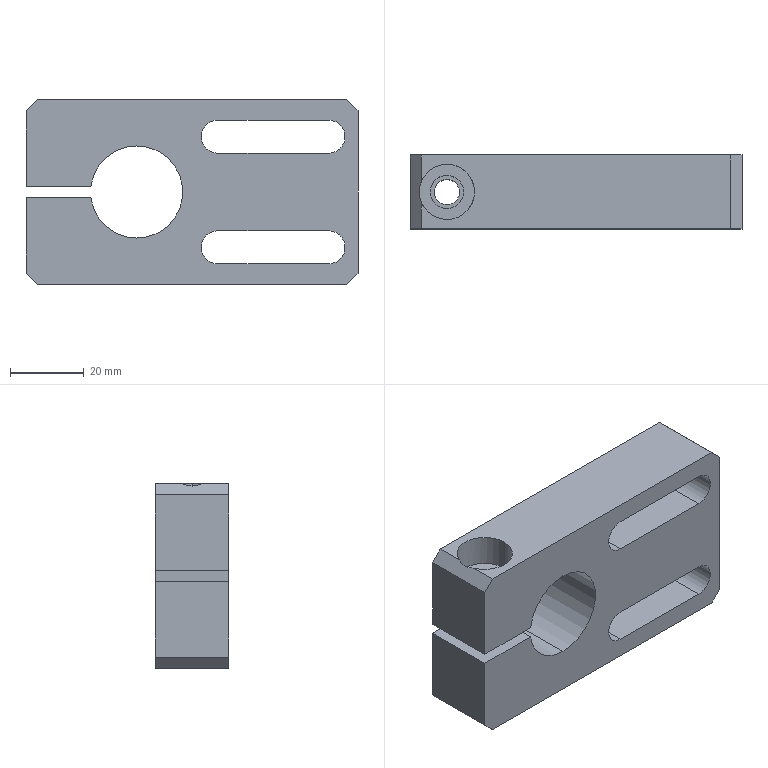Component | SolidWorks | 8TC-A15004-90-01A-1 | 1 solid | 31 faces | box 90 x 20 x 50 mm | volume 62105 mm3 | plane 18 | cylinder 13 | commonest cylinder face diameters 9 x6 25 x3 6.8 x2 15 x2 | material A3
build123d program:
from build123d import *

# Parameters (mm, degrees)
SKETCH1_W                                       = 90
SKETCH1_H                                       = 50
BOSS_EXTRUDE1_DEPTH                             = 10
SKETCH2_R                                       = 12.5
CUT_EXTRUDE1_DEPTH                              = 56.227
CHAMFER1_SIZE                                   = 3
CUT_EXTRUDE2_DEPTH                              = 56.227
SKETCH4_W                                       = 17.59
SKETCH4_H                                       = 3
CUT_EXTRUDE3_DEPTH                              = 56.227
M8_HEX_SOCKET_HEAD_CAP_SCREW_CBORE1_D           = 9
M8_HEX_SOCKET_HEAD_CAP_SCREW_CBORE1_DEPTH       = 23.5
M8_HEX_SOCKET_HEAD_CAP_SCREW_CBORE1_CBORE_D     = 15
M8_HEX_SOCKET_HEAD_CAP_SCREW_CBORE1_CBORE_DEPTH = 8.6
M8_TAPPED_HOLE1_D                               = 6.8


with BuildPart() as part:
    # Sketch1 → Boss-Extrude1 (new, symmetric)
    with BuildSketch(Plane(origin=(0, 0, 0), x_dir=(1, 0, 0), z_dir=(0, 1, 0))):
        Rectangle(SKETCH1_W, SKETCH1_H)
    extrude(amount=BOSS_EXTRUDE1_DEPTH, both=True)

    # Sketch2 → Cut-Extrude1 (cut, through all)
    with BuildSketch(Plane(origin=(0, 10, 0), x_dir=(1, 0, 0), z_dir=(0, 1, 0))):
        with Locations(Location((-15, 0, 0), (0, 0, 270))):
            Circle(SKETCH2_R)
    extrude(amount=-CUT_EXTRUDE1_DEPTH, mode=Mode.SUBTRACT)

    # Chamfer1
    chamfer1_edges = [part.edges().sort_by_distance(p)[0] for p in [
        (45, 0, 25),
        (-45, 0, 25),
        (-45, 0, -25),
        (45, 0, -25),
    ]]
    chamfer(chamfer1_edges, length=CHAMFER1_SIZE)

    # Sketch3 → Cut-Extrude2 (cut, through all)
    with BuildSketch(Plane(origin=(0, 10, 0), x_dir=(1, 0, 0), z_dir=(0, 1, 0))):
        with BuildLine():
            Line((7, 19.5), (37, 19.5))
            ThreePointArc((37, 19.5), (41.5, 15), (37, 10.5))
            Line((37, 10.5), (7, 10.5))
            ThreePointArc((7, 10.5), (2.5, 15), (7, 19.5))
        make_face()
        with BuildLine():
            Line((7, -19.5), (37, -19.5))
            ThreePointArc((37, -19.5), (41.5, -15), (37, -10.5))
            Line((37, -10.5), (7, -10.5))
            ThreePointArc((7, -10.5), (2.5, -15), (7, -19.5))
        make_face()
    extrude(amount=-CUT_EXTRUDE2_DEPTH, mode=Mode.SUBTRACT)

    # Sketch4 → Cut-Extrude3 (cut, through all)
    with BuildSketch(Plane(origin=(0, 10, 0), x_dir=(1, 0, 0), z_dir=(0, 1, 0))):
        with Locations((-36.205, 0)):
            Rectangle(SKETCH4_W, SKETCH4_H)
    extrude(amount=-CUT_EXTRUDE3_DEPTH, mode=Mode.SUBTRACT)

    # M8 Hex Socket Head Cap Screw CBORE1
    with Locations(Plane.XY.offset(25)):
        with Locations((-35, 0)):
            CounterBoreHole(M8_HEX_SOCKET_HEAD_CAP_SCREW_CBORE1_D / 2, M8_HEX_SOCKET_HEAD_CAP_SCREW_CBORE1_CBORE_D / 2, M8_HEX_SOCKET_HEAD_CAP_SCREW_CBORE1_CBORE_DEPTH, depth=M8_HEX_SOCKET_HEAD_CAP_SCREW_CBORE1_DEPTH)

    # M8 Tapped Hole1 (through all)
    with Locations(Plane.XY.offset(-1.5)):
        with Locations((-35, 0)):
            Hole(M8_TAPPED_HOLE1_D / 2)


solid = part.part
STEP:
#1=COLOUR_RGB('',0.7922,0.8196,0.9333);
#2=FILL_AREA_STYLE_COLOUR('',#1);
#3=FILL_AREA_STYLE('',(#2));
#4=SURFACE_STYLE_FILL_AREA(#3);
#5=SURFACE_SIDE_STYLE('',(#4));
#6=SURFACE_STYLE_USAGE(.BOTH.,#5);
#7=PRESENTATION_STYLE_ASSIGNMENT((#6));
#8=CARTESIAN_POINT('',(-1.512,-0.,-0.9843));
#9=VERTEX_POINT('',#8);
#10=CARTESIAN_POINT('',(-1.244,-0.,-0.9843));
#11=VERTEX_POINT('',#10);
#12=CARTESIAN_POINT('',(-1.378,-0.,-0.9843));
#13=DIRECTION('',(0.,0.,1.));
#14=DIRECTION('',(1.,0.,0.));
#15=AXIS2_PLACEMENT_3D('',#12,#13,#14);
#16=CIRCLE('',#15,0.1339);
#17=EDGE_CURVE('',#9,#11,#16,.T.);
#18=ORIENTED_EDGE('',*,*,#17,.F.);
#19=CARTESIAN_POINT('',(-1.512,-0.,-0.05906));
#20=VERTEX_POINT('',#19);
#21=CARTESIAN_POINT('',(-1.512,-0.,-0.05906));
#22=DIRECTION('',(0.,0.,1.));
#23=VECTOR('',#22,39.37);
#24=LINE('',#21,#23);
#25=EDGE_CURVE('',#9,#20,#24,.T.);
#26=ORIENTED_EDGE('',*,*,#25,.T.);
#27=CARTESIAN_POINT('',(-1.244,-0.,-0.05906));
#28=VERTEX_POINT('',#27);
#29=CARTESIAN_POINT('',(-1.378,-0.,-0.05906));
#30=DIRECTION('',(0.,0.,1.));
#31=DIRECTION('',(1.,0.,0.));
#32=AXIS2_PLACEMENT_3D('',#29,#30,#31);
#33=CIRCLE('',#32,0.1339);
#34=EDGE_CURVE('',#20,#28,#33,.T.);
#35=ORIENTED_EDGE('',*,*,#34,.T.);
#36=CARTESIAN_POINT('',(-1.244,-0.,-0.05906));
#37=DIRECTION('',(0.,0.,1.));
#38=VECTOR('',#37,39.37);
#39=LINE('',#36,#38);
#40=EDGE_CURVE('',#11,#28,#39,.T.);
#41=ORIENTED_EDGE('',*,*,#40,.F.);
#42=EDGE_LOOP('',(#18,#26,#35,#41));
#43=FACE_OUTER_BOUND('',#42,.T.);
#44=CARTESIAN_POINT('',(-1.378,-0.,-0.05906));
#45=DIRECTION('',(0.,0.,1.));
#46=DIRECTION('',(1.,0.,0.));
#47=AXIS2_PLACEMENT_3D('',#44,#45,#46);
#48=CYLINDRICAL_SURFACE('',#47,0.1339);
#49=ADVANCED_FACE('',(#43),#48,.F.);
#50=CARTESIAN_POINT('',(-1.673,-0.,0.6457));
#51=VERTEX_POINT('',#50);
#52=CARTESIAN_POINT('',(-1.083,-0.,0.6457));
#53=VERTEX_POINT('',#52);
#54=CARTESIAN_POINT('',(-1.378,-0.,0.6457));
#55=DIRECTION('',(0.,0.,1.));
#56=DIRECTION('',(1.,0.,0.));
#57=AXIS2_PLACEMENT_3D('',#54,#55,#56);
#58=CIRCLE('',#57,0.2953);
#59=EDGE_CURVE('',#51,#53,#58,.T.);
#60=ORIENTED_EDGE('',*,*,#59,.F.);
#61=CARTESIAN_POINT('',(-1.673,-0.,0.9646));
#62=VERTEX_POINT('',#61);
#63=CARTESIAN_POINT('',(-1.673,-0.,0.9843));
#64=DIRECTION('',(0.,0.,1.));
#65=VECTOR('',#64,39.37);
#66=LINE('',#63,#65);
#67=EDGE_CURVE('',#51,#62,#66,.T.);
#68=ORIENTED_EDGE('',*,*,#67,.T.);
#69=CARTESIAN_POINT('',(-1.654,-0.106,0.9843));
#70=VERTEX_POINT('',#69);
#71=CARTESIAN_POINT('',(-1.673,-0.,0.9646));
#72=CARTESIAN_POINT('',(-1.673,-0.03635,0.9646));
#73=CARTESIAN_POINT('',(-1.667,-0.07208,0.9712));
#74=CARTESIAN_POINT('',(-1.654,-0.106,0.9843));
#75=(BOUNDED_CURVE()B_SPLINE_CURVE(3,(#71,#72,#73,#74),.UNSPECIFIED.,.F.,.T.)B_SPLINE_CURVE_WITH_KNOTS((4,4),(3.142,3.509),.UNSPECIFIED.)CURVE()GEOMETRIC_REPRESENTATION_ITEM()RATIONAL_B_SPLINE_CURVE((1.,0.9888,0.9888,1.))REPRESENTATION_ITEM(''));
#76=EDGE_CURVE('',#62,#70,#75,.T.);
#77=ORIENTED_EDGE('',*,*,#76,.T.);
#78=CARTESIAN_POINT('',(-1.083,-0.,0.9843));
#79=VERTEX_POINT('',#78);
#80=CARTESIAN_POINT('',(-1.378,-0.,0.9843));
#81=DIRECTION('',(0.,0.,1.));
#82=DIRECTION('',(1.,0.,0.));
#83=AXIS2_PLACEMENT_3D('',#80,#81,#82);
#84=CIRCLE('',#83,0.2953);
#85=EDGE_CURVE('',#70,#79,#84,.T.);
#86=ORIENTED_EDGE('',*,*,#85,.T.);
#87=CARTESIAN_POINT('',(-1.083,-0.,0.9843));
#88=DIRECTION('',(0.,0.,1.));
#89=VECTOR('',#88,39.37);
#90=LINE('',#87,#89);
#91=EDGE_CURVE('',#53,#79,#90,.T.);
#92=ORIENTED_EDGE('',*,*,#91,.F.);
#93=EDGE_LOOP('',(#60,#68,#77,#86,#92));
#94=FACE_OUTER_BOUND('',#93,.T.);
#95=CARTESIAN_POINT('',(-1.378,-0.,0.9843));
#96=DIRECTION('',(0.,0.,1.));
#97=DIRECTION('',(1.,0.,0.));
#98=AXIS2_PLACEMENT_3D('',#95,#96,#97);
#99=CYLINDRICAL_SURFACE('',#98,0.2953);
#100=ADVANCED_FACE('',(#94),#99,.F.);
#101=CARTESIAN_POINT('',(-1.555,-0.,0.05906));
#102=VERTEX_POINT('',#101);
#103=CARTESIAN_POINT('',(-1.201,-0.,0.05906));
#104=VERTEX_POINT('',#103);
#105=CARTESIAN_POINT('',(-1.378,-0.,0.05906));
#106=DIRECTION('',(0.,0.,1.));
#107=DIRECTION('',(1.,0.,-0.));
#108=AXIS2_PLACEMENT_3D('',#105,#106,#107);
#109=CIRCLE('',#108,0.1772);
#110=EDGE_CURVE('',#102,#104,#109,.T.);
#111=ORIENTED_EDGE('',*,*,#110,.F.);
#112=CARTESIAN_POINT('',(-1.555,-0.,0.6457));
#113=VERTEX_POINT('',#112);
#114=CARTESIAN_POINT('',(-1.555,-0.,0.9843));
#115=DIRECTION('',(0.,0.,1.));
#116=VECTOR('',#115,39.37);
#117=LINE('',#114,#116);
#118=EDGE_CURVE('',#102,#113,#117,.T.);
#119=ORIENTED_EDGE('',*,*,#118,.T.);
#120=CARTESIAN_POINT('',(-1.201,-0.,0.6457));
#121=VERTEX_POINT('',#120);
#122=CARTESIAN_POINT('',(-1.378,-0.,0.6457));
#123=DIRECTION('',(0.,0.,1.));
#124=DIRECTION('',(1.,0.,0.));
#125=AXIS2_PLACEMENT_3D('',#122,#123,#124);
#126=CIRCLE('',#125,0.1772);
#127=EDGE_CURVE('',#113,#121,#126,.T.);
#128=ORIENTED_EDGE('',*,*,#127,.T.);
#129=CARTESIAN_POINT('',(-1.201,-0.,0.9843));
#130=DIRECTION('',(0.,0.,1.));
#131=VECTOR('',#130,39.37);
#132=LINE('',#129,#131);
#133=EDGE_CURVE('',#104,#121,#132,.T.);
#134=ORIENTED_EDGE('',*,*,#133,.F.);
#135=EDGE_LOOP('',(#111,#119,#128,#134));
#136=FACE_OUTER_BOUND('',#135,.T.);
#137=CARTESIAN_POINT('',(-1.378,-0.,0.9843));
#138=DIRECTION('',(0.,0.,1.));
#139=DIRECTION('',(1.,0.,0.));
#140=AXIS2_PLACEMENT_3D('',#137,#138,#139);
#141=CYLINDRICAL_SURFACE('',#140,0.1772);
#142=ADVANCED_FACE('',(#136),#141,.F.);
#143=CARTESIAN_POINT('',(-0.5906,-0.3937,-0.4921));
#144=VERTEX_POINT('',#143);
#145=CARTESIAN_POINT('',(-1.079,-0.3937,-0.05906));
#146=VERTEX_POINT('',#145);
#147=CARTESIAN_POINT('',(-0.5906,-0.3937,0.));
#148=DIRECTION('',(0.,1.,0.));
#149=DIRECTION('',(0.,0.,1.));
#150=AXIS2_PLACEMENT_3D('',#147,#148,#149);
#151=CIRCLE('',#150,0.4921);
#152=EDGE_CURVE('',#144,#146,#151,.T.);
#153=ORIENTED_EDGE('',*,*,#152,.F.);
#154=CARTESIAN_POINT('',(-0.5906,0.3937,-0.4921));
#155=VERTEX_POINT('',#154);
#156=CARTESIAN_POINT('',(-0.5906,-0.3937,-0.4921));
#157=DIRECTION('',(0.,1.,0.));
#158=VECTOR('',#157,39.37);
#159=LINE('',#156,#158);
#160=EDGE_CURVE('',#144,#155,#159,.T.);
#161=ORIENTED_EDGE('',*,*,#160,.T.);
#162=CARTESIAN_POINT('',(-1.079,0.3937,-0.05906));
#163=VERTEX_POINT('',#162);
#164=CARTESIAN_POINT('',(-0.5906,0.3937,0.));
#165=DIRECTION('',(0.,1.,0.));
#166=DIRECTION('',(0.,0.,1.));
#167=AXIS2_PLACEMENT_3D('',#164,#165,#166);
#168=CIRCLE('',#167,0.4921);
#169=EDGE_CURVE('',#155,#163,#168,.T.);
#170=ORIENTED_EDGE('',*,*,#169,.T.);
#171=CARTESIAN_POINT('',(-1.079,-0.3937,-0.05906));
#172=DIRECTION('',(0.,1.,0.));
#173=VECTOR('',#172,39.37);
#174=LINE('',#171,#173);
#175=EDGE_CURVE('',#146,#163,#174,.T.);
#176=ORIENTED_EDGE('',*,*,#175,.F.);
#177=EDGE_LOOP('',(#153,#161,#170,#176));
#178=FACE_OUTER_BOUND('',#177,.T.);
#179=CARTESIAN_POINT('',(-0.5906,-0.3937,0.));
#180=DIRECTION('',(0.,1.,0.));
#181=DIRECTION('',(0.,0.,1.));
#182=AXIS2_PLACEMENT_3D('',#179,#180,#181);
#183=CYLINDRICAL_SURFACE('',#182,0.4921);
#184=ADVANCED_FACE('',(#178),#183,.F.);
#185=ORIENTED_EDGE('',*,*,#160,.F.);
#186=CARTESIAN_POINT('',(-0.5906,-0.3937,0.4921));
#187=VERTEX_POINT('',#186);
#188=CARTESIAN_POINT('',(-0.5906,-0.3937,0.));
#189=DIRECTION('',(0.,1.,0.));
#190=DIRECTION('',(0.,0.,1.));
#191=AXIS2_PLACEMENT_3D('',#188,#189,#190);
#192=CIRCLE('',#191,0.4921);
#193=EDGE_CURVE('',#187,#144,#192,.T.);
#194=ORIENTED_EDGE('',*,*,#193,.F.);
#195=CARTESIAN_POINT('',(-0.5906,0.3937,0.4921));
#196=VERTEX_POINT('',#195);
#197=CARTESIAN_POINT('',(-0.5906,-0.3937,0.4921));
#198=DIRECTION('',(0.,1.,0.));
#199=VECTOR('',#198,39.37);
#200=LINE('',#197,#199);
#201=EDGE_CURVE('',#187,#196,#200,.T.);
#202=ORIENTED_EDGE('',*,*,#201,.T.);
#203=CARTESIAN_POINT('',(-0.5906,0.3937,0.));
#204=DIRECTION('',(0.,1.,0.));
#205=DIRECTION('',(0.,0.,1.));
#206=AXIS2_PLACEMENT_3D('',#203,#204,#205);
#207=CIRCLE('',#206,0.4921);
#208=EDGE_CURVE('',#196,#155,#207,.T.);
#209=ORIENTED_EDGE('',*,*,#208,.T.);
#210=EDGE_LOOP('',(#185,#194,#202,#209));
#211=FACE_OUTER_BOUND('',#210,.T.);
#212=CARTESIAN_POINT('',(-0.5906,-0.3937,0.));
#213=DIRECTION('',(0.,1.,0.));
#214=DIRECTION('',(0.,0.,1.));
#215=AXIS2_PLACEMENT_3D('',#212,#213,#214);
#216=CYLINDRICAL_SURFACE('',#215,0.4921);
#217=ADVANCED_FACE('',(#211),#216,.F.);
#218=ORIENTED_EDGE('',*,*,#85,.F.);
#219=CARTESIAN_POINT('',(-1.654,-0.3937,0.9843));
#220=VERTEX_POINT('',#219);
#221=CARTESIAN_POINT('',(-1.654,0.3937,0.9843));
#222=DIRECTION('',(0.,-1.,0.));
#223=VECTOR('',#222,39.37);
#224=LINE('',#221,#223);
#225=EDGE_CURVE('',#70,#220,#224,.T.);
#226=ORIENTED_EDGE('',*,*,#225,.T.);
#227=CARTESIAN_POINT('',(1.654,-0.3937,0.9843));
#228=VERTEX_POINT('',#227);
#229=CARTESIAN_POINT('',(-1.772,-0.3937,0.9843));
#230=DIRECTION('',(1.,0.,0.));
#231=VECTOR('',#230,39.37);
#232=LINE('',#229,#231);
#233=EDGE_CURVE('',#220,#228,#232,.T.);
#234=ORIENTED_EDGE('',*,*,#233,.T.);
#235=CARTESIAN_POINT('',(1.654,0.3937,0.9843));
#236=VERTEX_POINT('',#235);
#237=CARTESIAN_POINT('',(1.654,0.3937,0.9843));
#238=DIRECTION('',(0.,1.,0.));
#239=VECTOR('',#238,39.37);
#240=LINE('',#237,#239);
#241=EDGE_CURVE('',#228,#236,#240,.T.);
#242=ORIENTED_EDGE('',*,*,#241,.T.);
#243=CARTESIAN_POINT('',(-1.654,0.3937,0.9843));
#244=VERTEX_POINT('',#243);
#245=CARTESIAN_POINT('',(-1.772,0.3937,0.9843));
#246=DIRECTION('',(1.,0.,0.));
#247=VECTOR('',#246,39.37);
#248=LINE('',#245,#247);
#249=EDGE_CURVE('',#244,#236,#248,.T.);
#250=ORIENTED_EDGE('',*,*,#249,.F.);
#251=CARTESIAN_POINT('',(-1.654,0.106,0.9843));
#252=VERTEX_POINT('',#251);
#253=CARTESIAN_POINT('',(-1.654,0.3937,0.9843));
#254=DIRECTION('',(0.,-1.,0.));
#255=VECTOR('',#254,39.37);
#256=LINE('',#253,#255);
#257=EDGE_CURVE('',#244,#252,#256,.T.);
#258=ORIENTED_EDGE('',*,*,#257,.T.);
#259=CARTESIAN_POINT('',(-1.378,-0.,0.9843));
#260=DIRECTION('',(0.,0.,1.));
#261=DIRECTION('',(1.,0.,0.));
#262=AXIS2_PLACEMENT_3D('',#259,#260,#261);
#263=CIRCLE('',#262,0.2953);
#264=EDGE_CURVE('',#79,#252,#263,.T.);
#265=ORIENTED_EDGE('',*,*,#264,.F.);
#266=EDGE_LOOP('',(#218,#226,#234,#242,#250,#258,#265));
#267=FACE_OUTER_BOUND('',#266,.T.);
#268=CARTESIAN_POINT('',(-1.772,0.3937,0.9843));
#269=DIRECTION('',(0.,0.,-1.));
#270=DIRECTION('',(-1.,0.,0.));
#271=AXIS2_PLACEMENT_3D('',#268,#269,#270);
#272=PLANE('',#271);
#273=ADVANCED_FACE('',(#267),#272,.F.);
#274=CARTESIAN_POINT('',(-1.772,0.3937,0.05906));
#275=VERTEX_POINT('',#274);
#276=CARTESIAN_POINT('',(-1.772,0.3937,0.8661));
#277=VERTEX_POINT('',#276);
#278=CARTESIAN_POINT('',(-1.772,0.3937,0.9843));
#279=DIRECTION('',(0.,0.,1.));
#280=VECTOR('',#279,39.37);
#281=LINE('',#278,#280);
#282=EDGE_CURVE('',#275,#277,#281,.T.);
#283=ORIENTED_EDGE('',*,*,#282,.F.);
#284=CARTESIAN_POINT('',(-1.772,-0.3937,0.05906));
#285=VERTEX_POINT('',#284);
#286=CARTESIAN_POINT('',(-1.772,-0.3937,0.05906));
#287=DIRECTION('',(0.,1.,0.));
#288=VECTOR('',#287,39.37);
#289=LINE('',#286,#288);
#290=EDGE_CURVE('',#285,#275,#289,.T.);
#291=ORIENTED_EDGE('',*,*,#290,.F.);
#292=CARTESIAN_POINT('',(-1.772,-0.3937,0.8661));
#293=VERTEX_POINT('',#292);
#294=CARTESIAN_POINT('',(-1.772,-0.3937,0.9843));
#295=DIRECTION('',(0.,0.,1.));
#296=VECTOR('',#295,39.37);
#297=LINE('',#294,#296);
#298=EDGE_CURVE('',#285,#293,#297,.T.);
#299=ORIENTED_EDGE('',*,*,#298,.T.);
#300=CARTESIAN_POINT('',(-1.772,0.3937,0.8661));
#301=DIRECTION('',(0.,1.,0.));
#302=VECTOR('',#301,39.37);
#303=LINE('',#300,#302);
#304=EDGE_CURVE('',#293,#277,#303,.T.);
#305=ORIENTED_EDGE('',*,*,#304,.T.);
#306=EDGE_LOOP('',(#283,#291,#299,#305));
#307=FACE_OUTER_BOUND('',#306,.T.);
#308=CARTESIAN_POINT('',(-1.772,0.3937,0.9843));
#309=DIRECTION('',(1.,0.,0.));
#310=DIRECTION('',(0.,0.,-1.));
#311=AXIS2_PLACEMENT_3D('',#308,#309,#310);
#312=PLANE('',#311);
#313=ADVANCED_FACE('',(#307),#312,.F.);
#314=CARTESIAN_POINT('',(1.772,-0.3937,0.8661));
#315=VERTEX_POINT('',#314);
#316=CARTESIAN_POINT('',(1.772,-0.3937,-0.8661));
#317=VERTEX_POINT('',#316);
#318=CARTESIAN_POINT('',(1.772,-0.3937,0.9843));
#319=DIRECTION('',(0.,0.,-1.));
#320=VECTOR('',#319,39.37);
#321=LINE('',#318,#320);
#322=EDGE_CURVE('',#315,#317,#321,.T.);
#323=ORIENTED_EDGE('',*,*,#322,.T.);
#324=CARTESIAN_POINT('',(1.772,0.3937,-0.8661));
#325=VERTEX_POINT('',#324);
#326=CARTESIAN_POINT('',(1.772,0.3937,-0.8661));
#327=DIRECTION('',(0.,1.,0.));
#328=VECTOR('',#327,39.37);
#329=LINE('',#326,#328);
#330=EDGE_CURVE('',#317,#325,#329,.T.);
#331=ORIENTED_EDGE('',*,*,#330,.T.);
#332=CARTESIAN_POINT('',(1.772,0.3937,0.8661));
#333=VERTEX_POINT('',#332);
#334=CARTESIAN_POINT('',(1.772,0.3937,0.9843));
#335=DIRECTION('',(0.,0.,-1.));
#336=VECTOR('',#335,39.37);
#337=LINE('',#334,#336);
#338=EDGE_CURVE('',#333,#325,#337,.T.);
#339=ORIENTED_EDGE('',*,*,#338,.F.);
#340=CARTESIAN_POINT('',(1.772,0.3937,0.8661));
#341=DIRECTION('',(0.,-1.,0.));
#342=VECTOR('',#341,39.37);
#343=LINE('',#340,#342);
#344=EDGE_CURVE('',#333,#315,#343,.T.);
#345=ORIENTED_EDGE('',*,*,#344,.T.);
#346=EDGE_LOOP('',(#323,#331,#339,#345));
#347=FACE_OUTER_BOUND('',#346,.T.);
#348=CARTESIAN_POINT('',(1.772,0.3937,0.9843));
#349=DIRECTION('',(-1.,0.,0.));
#350=DIRECTION('',(0.,0.,1.));
#351=AXIS2_PLACEMENT_3D('',#348,#349,#350);
#352=PLANE('',#351);
#353=ADVANCED_FACE('',(#347),#352,.F.);
#354=CARTESIAN_POINT('',(-1.378,-0.,-0.9843));
#355=DIRECTION('',(0.,0.,1.));
#356=DIRECTION('',(1.,0.,0.));
#357=AXIS2_PLACEMENT_3D('',#354,#355,#356);
#358=CIRCLE('',#357,0.1339);
#359=EDGE_CURVE('',#11,#9,#358,.T.);
#360=ORIENTED_EDGE('',*,*,#359,.T.);
#361=ORIENTED_EDGE('',*,*,#17,.T.);
#362=EDGE_LOOP('',(#360,#361));
#363=FACE_BOUND('',#362,.T.);
#364=CARTESIAN_POINT('',(1.654,0.3937,-0.9843));
#365=VERTEX_POINT('',#364);
#366=CARTESIAN_POINT('',(-1.654,0.3937,-0.9843));
#367=VERTEX_POINT('',#366);
#368=CARTESIAN_POINT('',(-1.772,0.3937,-0.9843));
#369=DIRECTION('',(-1.,0.,0.));
#370=VECTOR('',#369,39.37);
#371=LINE('',#368,#370);
#372=EDGE_CURVE('',#365,#367,#371,.T.);
#373=ORIENTED_EDGE('',*,*,#372,.F.);
#374=CARTESIAN_POINT('',(1.654,-0.3937,-0.9843));
#375=VERTEX_POINT('',#374);
#376=CARTESIAN_POINT('',(1.654,0.3937,-0.9843));
#377=DIRECTION('',(0.,-1.,0.));
#378=VECTOR('',#377,39.37);
#379=LINE('',#376,#378);
#380=EDGE_CURVE('',#365,#375,#379,.T.);
#381=ORIENTED_EDGE('',*,*,#380,.T.);
#382=CARTESIAN_POINT('',(-1.654,-0.3937,-0.9843));
#383=VERTEX_POINT('',#382);
#384=CARTESIAN_POINT('',(-1.772,-0.3937,-0.9843));
#385=DIRECTION('',(-1.,0.,0.));
#386=VECTOR('',#385,39.37);
#387=LINE('',#384,#386);
#388=EDGE_CURVE('',#375,#383,#387,.T.);
#389=ORIENTED_EDGE('',*,*,#388,.T.);
#390=CARTESIAN_POINT('',(-1.654,0.3937,-0.9843));
#391=DIRECTION('',(0.,1.,0.));
#392=VECTOR('',#391,39.37);
#393=LINE('',#390,#392);
#394=EDGE_CURVE('',#383,#367,#393,.T.);
#395=ORIENTED_EDGE('',*,*,#394,.T.);
#396=EDGE_LOOP('',(#373,#381,#389,#395));
#397=FACE_OUTER_BOUND('',#396,.T.);
#398=CARTESIAN_POINT('',(-1.772,0.3937,-0.9843));
#399=DIRECTION('',(0.,0.,1.));
#400=DIRECTION('',(1.,0.,0.));
#401=AXIS2_PLACEMENT_3D('',#398,#399,#400);
#402=PLANE('',#401);
#403=ADVANCED_FACE('',(#363,#397),#402,.F.);
#404=CARTESIAN_POINT('',(-1.772,-0.3937,-0.8661));
#405=VERTEX_POINT('',#404);
#406=CARTESIAN_POINT('',(-1.772,-0.3937,-0.05906));
#407=VERTEX_POINT('',#406);
#408=CARTESIAN_POINT('',(-1.772,-0.3937,0.9843));
#409=DIRECTION('',(0.,0.,1.));
#410=VECTOR('',#409,39.37);
#411=LINE('',#408,#410);
#412=EDGE_CURVE('',#405,#407,#411,.T.);
#413=ORIENTED_EDGE('',*,*,#412,.T.);
#414=CARTESIAN_POINT('',(-1.772,0.3937,-0.05906));
#415=VERTEX_POINT('',#414);
#416=CARTESIAN_POINT('',(-1.772,-0.3937,-0.05906));
#417=DIRECTION('',(0.,1.,0.));
#418=VECTOR('',#417,39.37);
#419=LINE('',#416,#418);
#420=EDGE_CURVE('',#407,#415,#419,.T.);
#421=ORIENTED_EDGE('',*,*,#420,.T.);
#422=CARTESIAN_POINT('',(-1.772,0.3937,-0.8661));
#423=VERTEX_POINT('',#422);
#424=CARTESIAN_POINT('',(-1.772,0.3937,0.9843));
#425=DIRECTION('',(0.,0.,1.));
#426=VECTOR('',#425,39.37);
#427=LINE('',#424,#426);
#428=EDGE_CURVE('',#423,#415,#427,.T.);
#429=ORIENTED_EDGE('',*,*,#428,.F.);
#430=CARTESIAN_POINT('',(-1.772,0.3937,-0.8661));
#431=DIRECTION('',(0.,-1.,0.));
#432=VECTOR('',#431,39.37);
#433=LINE('',#430,#432);
#434=EDGE_CURVE('',#423,#405,#433,.T.);
#435=ORIENTED_EDGE('',*,*,#434,.T.);
#436=EDGE_LOOP('',(#413,#421,#429,#435));
#437=FACE_OUTER_BOUND('',#436,.T.);
#438=CARTESIAN_POINT('',(-1.772,0.3937,0.9843));
#439=DIRECTION('',(1.,0.,0.));
#440=DIRECTION('',(0.,0.,-1.));
#441=AXIS2_PLACEMENT_3D('',#438,#439,#440);
#442=PLANE('',#441);
#443=ADVANCED_FACE('',(#437),#442,.F.);
#444=CARTESIAN_POINT('',(0.2756,0.3937,0.7677));
#445=VERTEX_POINT('',#444);
#446=CARTESIAN_POINT('',(1.457,0.3937,0.7677));
#447=VERTEX_POINT('',#446);
#448=CARTESIAN_POINT('',(0.2756,0.3937,0.7677));
#449=DIRECTION('',(1.,0.,0.));
#450=VECTOR('',#449,39.37);
#451=LINE('',#448,#450);
#452=EDGE_CURVE('',#445,#447,#451,.T.);
#453=ORIENTED_EDGE('',*,*,#452,.F.);
#454=CARTESIAN_POINT('',(0.2756,0.3937,0.4134));
#455=VERTEX_POINT('',#454);
#456=CARTESIAN_POINT('',(0.2756,0.3937,0.5906));
#457=DIRECTION('',(0.,1.,0.));
#458=DIRECTION('',(0.,0.,-1.));
#459=AXIS2_PLACEMENT_3D('',#456,#457,#458);
#460=CIRCLE('',#459,0.1772);
#461=EDGE_CURVE('',#455,#445,#460,.T.);
#462=ORIENTED_EDGE('',*,*,#461,.F.);
#463=CARTESIAN_POINT('',(1.457,0.3937,0.4134));
#464=VERTEX_POINT('',#463);
#465=CARTESIAN_POINT('',(0.2756,0.3937,0.4134));
#466=DIRECTION('',(-1.,0.,0.));
#467=VECTOR('',#466,39.37);
#468=LINE('',#465,#467);
#469=EDGE_CURVE('',#464,#455,#468,.T.);
#470=ORIENTED_EDGE('',*,*,#469,.F.);
#471=CARTESIAN_POINT('',(1.457,0.3937,0.5906));
#472=DIRECTION('',(0.,1.,0.));
#473=DIRECTION('',(0.,0.,-1.));
#474=AXIS2_PLACEMENT_3D('',#471,#472,#473);
#475=CIRCLE('',#474,0.1772);
#476=EDGE_CURVE('',#447,#464,#475,.T.);
#477=ORIENTED_EDGE('',*,*,#476,.F.);
#478=EDGE_LOOP('',(#453,#462,#470,#477));
#479=FACE_BOUND('',#478,.T.);
#480=CARTESIAN_POINT('',(0.2756,0.3937,-0.4134));
#481=VERTEX_POINT('',#480);
#482=CARTESIAN_POINT('',(1.457,0.3937,-0.4134));
#483=VERTEX_POINT('',#482);
#484=CARTESIAN_POINT('',(0.2756,0.3937,-0.4134));
#485=DIRECTION('',(1.,0.,0.));
#486=VECTOR('',#485,39.37);
#487=LINE('',#484,#486);
#488=EDGE_CURVE('',#481,#483,#487,.T.);
#489=ORIENTED_EDGE('',*,*,#488,.F.);
#490=CARTESIAN_POINT('',(0.2756,0.3937,-0.7677));
#491=VERTEX_POINT('',#490);
#492=CARTESIAN_POINT('',(0.2756,0.3937,-0.5906));
#493=DIRECTION('',(0.,1.,0.));
#494=DIRECTION('',(0.,0.,1.));
#495=AXIS2_PLACEMENT_3D('',#492,#493,#494);
#496=CIRCLE('',#495,0.1772);
#497=EDGE_CURVE('',#491,#481,#496,.T.);
#498=ORIENTED_EDGE('',*,*,#497,.F.);
#499=CARTESIAN_POINT('',(1.457,0.3937,-0.7677));
#500=VERTEX_POINT('',#499);
#501=CARTESIAN_POINT('',(0.2756,0.3937,-0.7677));
#502=DIRECTION('',(-1.,0.,0.));
#503=VECTOR('',#502,39.37);
#504=LINE('',#501,#503);
#505=EDGE_CURVE('',#500,#491,#504,.T.);
#506=ORIENTED_EDGE('',*,*,#505,.F.);
#507=CARTESIAN_POINT('',(1.457,0.3937,-0.5906));
#508=DIRECTION('',(0.,1.,0.));
#509=DIRECTION('',(0.,0.,1.));
#510=AXIS2_PLACEMENT_3D('',#507,#508,#509);
#511=CIRCLE('',#510,0.1772);
#512=EDGE_CURVE('',#483,#500,#511,.T.);
#513=ORIENTED_EDGE('',*,*,#512,.F.);
#514=EDGE_LOOP('',(#489,#498,#506,#513));
#515=FACE_BOUND('',#514,.T.);
#516=CARTESIAN_POINT('',(-1.079,0.3937,0.05906));
#517=VERTEX_POINT('',#516);
#518=CARTESIAN_POINT('',(-0.5906,0.3937,0.));
#519=DIRECTION('',(0.,1.,0.));
#520=DIRECTION('',(0.,0.,1.));
#521=AXIS2_PLACEMENT_3D('',#518,#519,#520);
#522=CIRCLE('',#521,0.4921);
#523=EDGE_CURVE('',#517,#196,#522,.T.);
#524=ORIENTED_EDGE('',*,*,#523,.F.);
#525=CARTESIAN_POINT('',(-1.079,0.3937,0.05906));
#526=DIRECTION('',(1.,0.,-0.));
#527=VECTOR('',#526,39.37);
#528=LINE('',#525,#527);
#529=EDGE_CURVE('',#275,#517,#528,.T.);
#530=ORIENTED_EDGE('',*,*,#529,.F.);
#531=ORIENTED_EDGE('',*,*,#282,.T.);
#532=CARTESIAN_POINT('',(-1.654,0.3937,0.9843));
#533=DIRECTION('',(0.7071,0.,0.7071));
#534=VECTOR('',#533,39.37);
#535=LINE('',#532,#534);
#536=EDGE_CURVE('',#277,#244,#535,.T.);
#537=ORIENTED_EDGE('',*,*,#536,.T.);
#538=ORIENTED_EDGE('',*,*,#249,.T.);
#539=CARTESIAN_POINT('',(1.772,0.3937,0.8661));
#540=DIRECTION('',(0.7071,0.,-0.7071));
#541=VECTOR('',#540,39.37);
#542=LINE('',#539,#541);
#543=EDGE_CURVE('',#236,#333,#542,.T.);
#544=ORIENTED_EDGE('',*,*,#543,.T.);
#545=ORIENTED_EDGE('',*,*,#338,.T.);
#546=CARTESIAN_POINT('',(1.654,0.3937,-0.9843));
#547=DIRECTION('',(-0.7071,0.,-0.7071));
#548=VECTOR('',#547,39.37);
#549=LINE('',#546,#548);
#550=EDGE_CURVE('',#325,#365,#549,.T.);
#551=ORIENTED_EDGE('',*,*,#550,.T.);
#552=ORIENTED_EDGE('',*,*,#372,.T.);
#553=CARTESIAN_POINT('',(-1.772,0.3937,-0.8661));
#554=DIRECTION('',(-0.7071,0.,0.7071));
#555=VECTOR('',#554,39.37);
#556=LINE('',#553,#555);
#557=EDGE_CURVE('',#367,#423,#556,.T.);
#558=ORIENTED_EDGE('',*,*,#557,.T.);
#559=ORIENTED_EDGE('',*,*,#428,.T.);
#560=CARTESIAN_POINT('',(-1.079,0.3937,-0.05906));
#561=DIRECTION('',(-1.,0.,-0.));
#562=VECTOR('',#561,39.37);
#563=LINE('',#560,#562);
#564=EDGE_CURVE('',#163,#415,#563,.T.);
#565=ORIENTED_EDGE('',*,*,#564,.F.);
#566=ORIENTED_EDGE('',*,*,#169,.F.);
#567=ORIENTED_EDGE('',*,*,#208,.F.);
#568=EDGE_LOOP('',(#524,#530,#531,#537,#538,#544,#545,#551,#552,#558,#559,#565,#566,#567));
#569=FACE_OUTER_BOUND('',#568,.T.);
#570=CARTESIAN_POINT('',(0.,0.3937,0.));
#571=DIRECTION('',(0.,-1.,0.));
#572=DIRECTION('',(0.,0.,-1.));
#573=AXIS2_PLACEMENT_3D('',#570,#571,#572);
#574=PLANE('',#573);
#575=ADVANCED_FACE('',(#479,#515,#569),#574,.F.);
#576=CARTESIAN_POINT('',(-1.079,-0.3937,0.05906));
#577=VERTEX_POINT('',#576);
#578=CARTESIAN_POINT('',(-1.079,-0.3937,0.05906));
#579=DIRECTION('',(1.,0.,-0.));
#580=VECTOR('',#579,39.37);
#581=LINE('',#578,#580);
#582=EDGE_CURVE('',#285,#577,#581,.T.);
#583=ORIENTED_EDGE('',*,*,#582,.T.);
#584=CARTESIAN_POINT('',(-0.5906,-0.3937,0.));
#585=DIRECTION('',(0.,1.,0.));
#586=DIRECTION('',(0.,0.,1.));
#587=AXIS2_PLACEMENT_3D('',#584,#585,#586);
#588=CIRCLE('',#587,0.4921);
#589=EDGE_CURVE('',#577,#187,#588,.T.);
#590=ORIENTED_EDGE('',*,*,#589,.T.);
#591=ORIENTED_EDGE('',*,*,#193,.T.);
#592=ORIENTED_EDGE('',*,*,#152,.T.);
#593=CARTESIAN_POINT('',(-1.079,-0.3937,-0.05906));
#594=DIRECTION('',(-1.,0.,-0.));
#595=VECTOR('',#594,39.37);
#596=LINE('',#593,#595);
#597=EDGE_CURVE('',#146,#407,#596,.T.);
#598=ORIENTED_EDGE('',*,*,#597,.T.);
#599=ORIENTED_EDGE('',*,*,#412,.F.);
#600=CARTESIAN_POINT('',(-1.319,-0.3937,-1.319));
#601=DIRECTION('',(0.7071,0.,-0.7071));
#602=VECTOR('',#601,39.37);
#603=LINE('',#600,#602);
#604=EDGE_CURVE('',#405,#383,#603,.T.);
#605=ORIENTED_EDGE('',*,*,#604,.T.);
#606=ORIENTED_EDGE('',*,*,#388,.F.);
#607=CARTESIAN_POINT('',(1.319,-0.3937,-1.319));
#608=DIRECTION('',(0.7071,0.,0.7071));
#609=VECTOR('',#608,39.37);
#610=LINE('',#607,#609);
#611=EDGE_CURVE('',#375,#317,#610,.T.);
#612=ORIENTED_EDGE('',*,*,#611,.T.);
#613=ORIENTED_EDGE('',*,*,#322,.F.);
#614=CARTESIAN_POINT('',(1.319,-0.3937,1.319));
#615=DIRECTION('',(-0.7071,0.,0.7071));
#616=VECTOR('',#615,39.37);
#617=LINE('',#614,#616);
#618=EDGE_CURVE('',#315,#228,#617,.T.);
#619=ORIENTED_EDGE('',*,*,#618,.T.);
#620=ORIENTED_EDGE('',*,*,#233,.F.);
#621=CARTESIAN_POINT('',(-1.319,-0.3937,1.319));
#622=DIRECTION('',(-0.7071,0.,-0.7071));
#623=VECTOR('',#622,39.37);
#624=LINE('',#621,#623);
#625=EDGE_CURVE('',#220,#293,#624,.T.);
#626=ORIENTED_EDGE('',*,*,#625,.T.);
#627=ORIENTED_EDGE('',*,*,#298,.F.);
#628=EDGE_LOOP('',(#583,#590,#591,#592,#598,#599,#605,#606,#612,#613,#619,#620,#626,#627));
#629=FACE_OUTER_BOUND('',#628,.T.);
#630=CARTESIAN_POINT('',(0.2756,-0.3937,0.4134));
#631=VERTEX_POINT('',#630);
#632=CARTESIAN_POINT('',(0.2756,-0.3937,0.7677));
#633=VERTEX_POINT('',#632);
#634=CARTESIAN_POINT('',(0.2756,-0.3937,0.5906));
#635=DIRECTION('',(0.,1.,0.));
#636=DIRECTION('',(0.,0.,-1.));
#637=AXIS2_PLACEMENT_3D('',#634,#635,#636);
#638=CIRCLE('',#637,0.1772);
#639=EDGE_CURVE('',#631,#633,#638,.T.);
#640=ORIENTED_EDGE('',*,*,#639,.T.);
#641=CARTESIAN_POINT('',(1.457,-0.3937,0.7677));
#642=VERTEX_POINT('',#641);
#643=CARTESIAN_POINT('',(0.2756,-0.3937,0.7677));
#644=DIRECTION('',(1.,0.,0.));
#645=VECTOR('',#644,39.37);
#646=LINE('',#643,#645);
#647=EDGE_CURVE('',#633,#642,#646,.T.);
#648=ORIENTED_EDGE('',*,*,#647,.T.);
#649=CARTESIAN_POINT('',(1.457,-0.3937,0.4134));
#650=VERTEX_POINT('',#649);
#651=CARTESIAN_POINT('',(1.457,-0.3937,0.5906));
#652=DIRECTION('',(0.,1.,0.));
#653=DIRECTION('',(0.,0.,-1.));
#654=AXIS2_PLACEMENT_3D('',#651,#652,#653);
#655=CIRCLE('',#654,0.1772);
#656=EDGE_CURVE('',#642,#650,#655,.T.);
#657=ORIENTED_EDGE('',*,*,#656,.T.);
#658=CARTESIAN_POINT('',(0.2756,-0.3937,0.4134));
#659=DIRECTION('',(-1.,0.,0.));
#660=VECTOR('',#659,39.37);
#661=LINE('',#658,#660);
#662=EDGE_CURVE('',#650,#631,#661,.T.);
#663=ORIENTED_EDGE('',*,*,#662,.T.);
#664=EDGE_LOOP('',(#640,#648,#657,#663));
#665=FACE_BOUND('',#664,.T.);
#666=CARTESIAN_POINT('',(0.2756,-0.3937,-0.7677));
#667=VERTEX_POINT('',#666);
#668=CARTESIAN_POINT('',(0.2756,-0.3937,-0.4134));
#669=VERTEX_POINT('',#668);
#670=CARTESIAN_POINT('',(0.2756,-0.3937,-0.5906));
#671=DIRECTION('',(0.,1.,0.));
#672=DIRECTION('',(0.,0.,1.));
#673=AXIS2_PLACEMENT_3D('',#670,#671,#672);
#674=CIRCLE('',#673,0.1772);
#675=EDGE_CURVE('',#667,#669,#674,.T.);
#676=ORIENTED_EDGE('',*,*,#675,.T.);
#677=CARTESIAN_POINT('',(1.457,-0.3937,-0.4134));
#678=VERTEX_POINT('',#677);
#679=CARTESIAN_POINT('',(0.2756,-0.3937,-0.4134));
#680=DIRECTION('',(1.,0.,0.));
#681=VECTOR('',#680,39.37);
#682=LINE('',#679,#681);
#683=EDGE_CURVE('',#669,#678,#682,.T.);
#684=ORIENTED_EDGE('',*,*,#683,.T.);
#685=CARTESIAN_POINT('',(1.457,-0.3937,-0.7677));
#686=VERTEX_POINT('',#685);
#687=CARTESIAN_POINT('',(1.457,-0.3937,-0.5906));
#688=DIRECTION('',(0.,1.,0.));
#689=DIRECTION('',(0.,0.,1.));
#690=AXIS2_PLACEMENT_3D('',#687,#688,#689);
#691=CIRCLE('',#690,0.1772);
#692=EDGE_CURVE('',#678,#686,#691,.T.);
#693=ORIENTED_EDGE('',*,*,#692,.T.);
#694=CARTESIAN_POINT('',(0.2756,-0.3937,-0.7677));
#695=DIRECTION('',(-1.,0.,0.));
#696=VECTOR('',#695,39.37);
#697=LINE('',#694,#696);
#698=EDGE_CURVE('',#686,#667,#697,.T.);
#699=ORIENTED_EDGE('',*,*,#698,.T.);
#700=EDGE_LOOP('',(#676,#684,#693,#699));
#701=FACE_BOUND('',#700,.T.);
#702=CARTESIAN_POINT('',(0.,-0.3937,0.));
#703=DIRECTION('',(0.,-1.,0.));
#704=DIRECTION('',(0.,0.,-1.));
#705=AXIS2_PLACEMENT_3D('',#702,#703,#704);
#706=PLANE('',#705);
#707=ADVANCED_FACE('',(#629,#665,#701),#706,.T.);
#708=ORIENTED_EDGE('',*,*,#201,.F.);
#709=ORIENTED_EDGE('',*,*,#589,.F.);
#710=CARTESIAN_POINT('',(-1.079,-0.3937,0.05906));
#711=DIRECTION('',(0.,1.,0.));
#712=VECTOR('',#711,39.37);
#713=LINE('',#710,#712);
#714=EDGE_CURVE('',#577,#517,#713,.T.);
#715=ORIENTED_EDGE('',*,*,#714,.T.);
#716=ORIENTED_EDGE('',*,*,#523,.T.);
#717=EDGE_LOOP('',(#708,#709,#715,#716));
#718=FACE_OUTER_BOUND('',#717,.T.);
#719=CARTESIAN_POINT('',(-0.5906,-0.3937,0.));
#720=DIRECTION('',(0.,1.,0.));
#721=DIRECTION('',(0.,0.,1.));
#722=AXIS2_PLACEMENT_3D('',#719,#720,#721);
#723=CYLINDRICAL_SURFACE('',#722,0.4921);
#724=ADVANCED_FACE('',(#718),#723,.F.);
#725=ORIENTED_EDGE('',*,*,#550,.F.);
#726=ORIENTED_EDGE('',*,*,#330,.F.);
#727=ORIENTED_EDGE('',*,*,#611,.F.);
#728=ORIENTED_EDGE('',*,*,#380,.F.);
#729=EDGE_LOOP('',(#725,#726,#727,#728));
#730=FACE_OUTER_BOUND('',#729,.T.);
#731=CARTESIAN_POINT('',(1.654,0.3937,-0.9843));
#732=DIRECTION('',(-0.7071,0.,0.7071));
#733=DIRECTION('',(0.,-1.,0.));
#734=AXIS2_PLACEMENT_3D('',#731,#732,#733);
#735=PLANE('',#734);
#736=ADVANCED_FACE('',(#730),#735,.F.);
#737=ORIENTED_EDGE('',*,*,#543,.F.);
#738=ORIENTED_EDGE('',*,*,#241,.F.);
#739=ORIENTED_EDGE('',*,*,#618,.F.);
#740=ORIENTED_EDGE('',*,*,#344,.F.);
#741=EDGE_LOOP('',(#737,#738,#739,#740));
#742=FACE_OUTER_BOUND('',#741,.T.);
#743=CARTESIAN_POINT('',(1.772,0.3937,0.8661));
#744=DIRECTION('',(-0.7071,0.,-0.7071));
#745=DIRECTION('',(0.,-1.,0.));
#746=AXIS2_PLACEMENT_3D('',#743,#744,#745);
#747=PLANE('',#746);
#748=ADVANCED_FACE('',(#742),#747,.F.);
#749=ORIENTED_EDGE('',*,*,#557,.F.);
#750=ORIENTED_EDGE('',*,*,#394,.F.);
#751=ORIENTED_EDGE('',*,*,#604,.F.);
#752=ORIENTED_EDGE('',*,*,#434,.F.);
#753=EDGE_LOOP('',(#749,#750,#751,#752));
#754=FACE_OUTER_BOUND('',#753,.T.);
#755=CARTESIAN_POINT('',(-1.772,0.3937,-0.8661));
#756=DIRECTION('',(0.7071,0.,0.7071));
#757=DIRECTION('',(0.,-1.,0.));
#758=AXIS2_PLACEMENT_3D('',#755,#756,#757);
#759=PLANE('',#758);
#760=ADVANCED_FACE('',(#754),#759,.F.);
#761=CARTESIAN_POINT('',(-1.654,0.106,0.9843));
#762=CARTESIAN_POINT('',(-1.667,0.07208,0.9712));
#763=CARTESIAN_POINT('',(-1.673,0.03635,0.9646));
#764=CARTESIAN_POINT('',(-1.673,-0.,0.9646));
#765=(BOUNDED_CURVE()B_SPLINE_CURVE(3,(#761,#762,#763,#764),.UNSPECIFIED.,.F.,.F.)B_SPLINE_CURVE_WITH_KNOTS((4,4),(2.774,3.142),.UNSPECIFIED.)CURVE()GEOMETRIC_REPRESENTATION_ITEM()RATIONAL_B_SPLINE_CURVE((1.,0.9888,0.9888,1.))REPRESENTATION_ITEM(''));
#766=EDGE_CURVE('',#252,#62,#765,.T.);
#767=ORIENTED_EDGE('',*,*,#766,.F.);
#768=ORIENTED_EDGE('',*,*,#257,.F.);
#769=ORIENTED_EDGE('',*,*,#536,.F.);
#770=ORIENTED_EDGE('',*,*,#304,.F.);
#771=ORIENTED_EDGE('',*,*,#625,.F.);
#772=ORIENTED_EDGE('',*,*,#225,.F.);
#773=ORIENTED_EDGE('',*,*,#76,.F.);
#774=EDGE_LOOP('',(#767,#768,#769,#770,#771,#772,#773));
#775=FACE_OUTER_BOUND('',#774,.T.);
#776=CARTESIAN_POINT('',(-1.654,0.3937,0.9843));
#777=DIRECTION('',(0.7071,0.,-0.7071));
#778=DIRECTION('',(0.,-1.,0.));
#779=AXIS2_PLACEMENT_3D('',#776,#777,#778);
#780=PLANE('',#779);
#781=ADVANCED_FACE('',(#775),#780,.F.);
#782=ORIENTED_EDGE('',*,*,#497,.T.);
#783=CARTESIAN_POINT('',(0.2756,-0.3937,-0.4134));
#784=DIRECTION('',(0.,1.,0.));
#785=VECTOR('',#784,39.37);
#786=LINE('',#783,#785);
#787=EDGE_CURVE('',#669,#481,#786,.T.);
#788=ORIENTED_EDGE('',*,*,#787,.F.);
#789=ORIENTED_EDGE('',*,*,#675,.F.);
#790=CARTESIAN_POINT('',(0.2756,-0.3937,-0.7677));
#791=DIRECTION('',(0.,1.,0.));
#792=VECTOR('',#791,39.37);
#793=LINE('',#790,#792);
#794=EDGE_CURVE('',#667,#491,#793,.T.);
#795=ORIENTED_EDGE('',*,*,#794,.T.);
#796=EDGE_LOOP('',(#782,#788,#789,#795));
#797=FACE_OUTER_BOUND('',#796,.T.);
#798=CARTESIAN_POINT('',(0.2756,-0.3937,-0.5906));
#799=DIRECTION('',(0.,1.,0.));
#800=DIRECTION('',(0.,0.,1.));
#801=AXIS2_PLACEMENT_3D('',#798,#799,#800);
#802=CYLINDRICAL_SURFACE('',#801,0.1772);
#803=ADVANCED_FACE('',(#797),#802,.F.);
#804=ORIENTED_EDGE('',*,*,#505,.T.);
#805=ORIENTED_EDGE('',*,*,#794,.F.);
#806=ORIENTED_EDGE('',*,*,#698,.F.);
#807=CARTESIAN_POINT('',(1.457,-0.3937,-0.7677));
#808=DIRECTION('',(0.,1.,0.));
#809=VECTOR('',#808,39.37);
#810=LINE('',#807,#809);
#811=EDGE_CURVE('',#686,#500,#810,.T.);
#812=ORIENTED_EDGE('',*,*,#811,.T.);
#813=EDGE_LOOP('',(#804,#805,#806,#812));
#814=FACE_OUTER_BOUND('',#813,.T.);
#815=CARTESIAN_POINT('',(0.2756,-0.3937,-0.7677));
#816=DIRECTION('',(0.,0.,-1.));
#817=DIRECTION('',(-1.,0.,0.));
#818=AXIS2_PLACEMENT_3D('',#815,#816,#817);
#819=PLANE('',#818);
#820=ADVANCED_FACE('',(#814),#819,.F.);
#821=ORIENTED_EDGE('',*,*,#512,.T.);
#822=ORIENTED_EDGE('',*,*,#811,.F.);
#823=ORIENTED_EDGE('',*,*,#692,.F.);
#824=CARTESIAN_POINT('',(1.457,-0.3937,-0.4134));
#825=DIRECTION('',(0.,1.,0.));
#826=VECTOR('',#825,39.37);
#827=LINE('',#824,#826);
#828=EDGE_CURVE('',#678,#483,#827,.T.);
#829=ORIENTED_EDGE('',*,*,#828,.T.);
#830=EDGE_LOOP('',(#821,#822,#823,#829));
#831=FACE_OUTER_BOUND('',#830,.T.);
#832=CARTESIAN_POINT('',(1.457,-0.3937,-0.5906));
#833=DIRECTION('',(0.,1.,0.));
#834=DIRECTION('',(0.,0.,1.));
#835=AXIS2_PLACEMENT_3D('',#832,#833,#834);
#836=CYLINDRICAL_SURFACE('',#835,0.1772);
#837=ADVANCED_FACE('',(#831),#836,.F.);
#838=ORIENTED_EDGE('',*,*,#488,.T.);
#839=ORIENTED_EDGE('',*,*,#828,.F.);
#840=ORIENTED_EDGE('',*,*,#683,.F.);
#841=ORIENTED_EDGE('',*,*,#787,.T.);
#842=EDGE_LOOP('',(#838,#839,#840,#841));
#843=FACE_OUTER_BOUND('',#842,.T.);
#844=CARTESIAN_POINT('',(0.2756,-0.3937,-0.4134));
#845=DIRECTION('',(0.,0.,1.));
#846=DIRECTION('',(1.,0.,0.));
#847=AXIS2_PLACEMENT_3D('',#844,#845,#846);
#848=PLANE('',#847);
#849=ADVANCED_FACE('',(#843),#848,.F.);
#850=ORIENTED_EDGE('',*,*,#461,.T.);
#851=CARTESIAN_POINT('',(0.2756,-0.3937,0.7677));
#852=DIRECTION('',(0.,1.,0.));
#853=VECTOR('',#852,39.37);
#854=LINE('',#851,#853);
#855=EDGE_CURVE('',#633,#445,#854,.T.);
#856=ORIENTED_EDGE('',*,*,#855,.F.);
#857=ORIENTED_EDGE('',*,*,#639,.F.);
#858=CARTESIAN_POINT('',(0.2756,-0.3937,0.4134));
#859=DIRECTION('',(0.,1.,0.));
#860=VECTOR('',#859,39.37);
#861=LINE('',#858,#860);
#862=EDGE_CURVE('',#631,#455,#861,.T.);
#863=ORIENTED_EDGE('',*,*,#862,.T.);
#864=EDGE_LOOP('',(#850,#856,#857,#863));
#865=FACE_OUTER_BOUND('',#864,.T.);
#866=CARTESIAN_POINT('',(0.2756,-0.3937,0.5906));
#867=DIRECTION('',(0.,1.,0.));
#868=DIRECTION('',(0.,0.,1.));
#869=AXIS2_PLACEMENT_3D('',#866,#867,#868);
#870=CYLINDRICAL_SURFACE('',#869,0.1772);
#871=ADVANCED_FACE('',(#865),#870,.F.);
#872=ORIENTED_EDGE('',*,*,#469,.T.);
#873=ORIENTED_EDGE('',*,*,#862,.F.);
#874=ORIENTED_EDGE('',*,*,#662,.F.);
#875=CARTESIAN_POINT('',(1.457,-0.3937,0.4134));
#876=DIRECTION('',(0.,1.,0.));
#877=VECTOR('',#876,39.37);
#878=LINE('',#875,#877);
#879=EDGE_CURVE('',#650,#464,#878,.T.);
#880=ORIENTED_EDGE('',*,*,#879,.T.);
#881=EDGE_LOOP('',(#872,#873,#874,#880));
#882=FACE_OUTER_BOUND('',#881,.T.);
#883=CARTESIAN_POINT('',(0.2756,-0.3937,0.4134));
#884=DIRECTION('',(0.,0.,-1.));
#885=DIRECTION('',(-1.,0.,0.));
#886=AXIS2_PLACEMENT_3D('',#883,#884,#885);
#887=PLANE('',#886);
#888=ADVANCED_FACE('',(#882),#887,.F.);
#889=ORIENTED_EDGE('',*,*,#476,.T.);
#890=ORIENTED_EDGE('',*,*,#879,.F.);
#891=ORIENTED_EDGE('',*,*,#656,.F.);
#892=CARTESIAN_POINT('',(1.457,-0.3937,0.7677));
#893=DIRECTION('',(0.,1.,0.));
#894=VECTOR('',#893,39.37);
#895=LINE('',#892,#894);
#896=EDGE_CURVE('',#642,#447,#895,.T.);
#897=ORIENTED_EDGE('',*,*,#896,.T.);
#898=EDGE_LOOP('',(#889,#890,#891,#897));
#899=FACE_OUTER_BOUND('',#898,.T.);
#900=CARTESIAN_POINT('',(1.457,-0.3937,0.5906));
#901=DIRECTION('',(0.,1.,0.));
#902=DIRECTION('',(0.,0.,1.));
#903=AXIS2_PLACEMENT_3D('',#900,#901,#902);
#904=CYLINDRICAL_SURFACE('',#903,0.1772);
#905=ADVANCED_FACE('',(#899),#904,.F.);
#906=ORIENTED_EDGE('',*,*,#452,.T.);
#907=ORIENTED_EDGE('',*,*,#896,.F.);
#908=ORIENTED_EDGE('',*,*,#647,.F.);
#909=ORIENTED_EDGE('',*,*,#855,.T.);
#910=EDGE_LOOP('',(#906,#907,#908,#909));
#911=FACE_OUTER_BOUND('',#910,.T.);
#912=CARTESIAN_POINT('',(0.2756,-0.3937,0.7677));
#913=DIRECTION('',(0.,0.,1.));
#914=DIRECTION('',(1.,0.,0.));
#915=AXIS2_PLACEMENT_3D('',#912,#913,#914);
#916=PLANE('',#915);
#917=ADVANCED_FACE('',(#911),#916,.F.);
#918=CARTESIAN_POINT('',(-1.378,-0.,-0.05906));
#919=DIRECTION('',(0.,0.,1.));
#920=DIRECTION('',(1.,0.,0.));
#921=AXIS2_PLACEMENT_3D('',#918,#919,#920);
#922=CIRCLE('',#921,0.1339);
#923=EDGE_CURVE('',#28,#20,#922,.T.);
#924=ORIENTED_EDGE('',*,*,#923,.F.);
#925=ORIENTED_EDGE('',*,*,#34,.F.);
#926=EDGE_LOOP('',(#924,#925));
#927=FACE_BOUND('',#926,.T.);
#928=ORIENTED_EDGE('',*,*,#564,.T.);
#929=ORIENTED_EDGE('',*,*,#420,.F.);
#930=ORIENTED_EDGE('',*,*,#597,.F.);
#931=ORIENTED_EDGE('',*,*,#175,.T.);
#932=EDGE_LOOP('',(#928,#929,#930,#931));
#933=FACE_OUTER_BOUND('',#932,.T.);
#934=CARTESIAN_POINT('',(-1.079,-0.3937,-0.05906));
#935=DIRECTION('',(0.,0.,-1.));
#936=DIRECTION('',(-1.,0.,-0.));
#937=AXIS2_PLACEMENT_3D('',#934,#935,#936);
#938=PLANE('',#937);
#939=ADVANCED_FACE('',(#927,#933),#938,.F.);
#940=CARTESIAN_POINT('',(-1.378,-0.,0.05906));
#941=DIRECTION('',(0.,0.,1.));
#942=DIRECTION('',(1.,0.,-0.));
#943=AXIS2_PLACEMENT_3D('',#940,#941,#942);
#944=CIRCLE('',#943,0.1772);
#945=EDGE_CURVE('',#104,#102,#944,.T.);
#946=ORIENTED_EDGE('',*,*,#945,.T.);
#947=ORIENTED_EDGE('',*,*,#110,.T.);
#948=EDGE_LOOP('',(#946,#947));
#949=FACE_BOUND('',#948,.T.);
#950=ORIENTED_EDGE('',*,*,#529,.T.);
#951=ORIENTED_EDGE('',*,*,#714,.F.);
#952=ORIENTED_EDGE('',*,*,#582,.F.);
#953=ORIENTED_EDGE('',*,*,#290,.T.);
#954=EDGE_LOOP('',(#950,#951,#952,#953));
#955=FACE_OUTER_BOUND('',#954,.T.);
#956=CARTESIAN_POINT('',(-1.079,-0.3937,0.05906));
#957=DIRECTION('',(0.,0.,1.));
#958=DIRECTION('',(1.,0.,-0.));
#959=AXIS2_PLACEMENT_3D('',#956,#957,#958);
#960=PLANE('',#959);
#961=ADVANCED_FACE('',(#949,#955),#960,.F.);
#962=ORIENTED_EDGE('',*,*,#118,.F.);
#963=ORIENTED_EDGE('',*,*,#945,.F.);
#964=ORIENTED_EDGE('',*,*,#133,.T.);
#965=CARTESIAN_POINT('',(-1.378,-0.,0.6457));
#966=DIRECTION('',(0.,0.,1.));
#967=DIRECTION('',(1.,0.,0.));
#968=AXIS2_PLACEMENT_3D('',#965,#966,#967);
#969=CIRCLE('',#968,0.1772);
#970=EDGE_CURVE('',#121,#113,#969,.T.);
#971=ORIENTED_EDGE('',*,*,#970,.T.);
#972=EDGE_LOOP('',(#962,#963,#964,#971));
#973=FACE_OUTER_BOUND('',#972,.T.);
#974=CARTESIAN_POINT('',(-1.378,-0.,0.9843));
#975=DIRECTION('',(0.,0.,1.));
#976=DIRECTION('',(1.,0.,0.));
#977=AXIS2_PLACEMENT_3D('',#974,#975,#976);
#978=CYLINDRICAL_SURFACE('',#977,0.1772);
#979=ADVANCED_FACE('',(#973),#978,.F.);
#980=ORIENTED_EDGE('',*,*,#970,.F.);
#981=ORIENTED_EDGE('',*,*,#127,.F.);
#982=EDGE_LOOP('',(#980,#981));
#983=FACE_BOUND('',#982,.T.);
#984=CARTESIAN_POINT('',(-1.378,-0.,0.6457));
#985=DIRECTION('',(0.,0.,1.));
#986=DIRECTION('',(1.,0.,0.));
#987=AXIS2_PLACEMENT_3D('',#984,#985,#986);
#988=CIRCLE('',#987,0.2953);
#989=EDGE_CURVE('',#53,#51,#988,.T.);
#990=ORIENTED_EDGE('',*,*,#989,.T.);
#991=ORIENTED_EDGE('',*,*,#59,.T.);
#992=EDGE_LOOP('',(#990,#991));
#993=FACE_OUTER_BOUND('',#992,.T.);
#994=CARTESIAN_POINT('',(-1.201,-0.,0.6457));
#995=DIRECTION('',(0.,0.,-1.));
#996=DIRECTION('',(-1.,0.,0.));
#997=AXIS2_PLACEMENT_3D('',#994,#995,#996);
#998=PLANE('',#997);
#999=ADVANCED_FACE('',(#983,#993),#998,.F.);
#1000=ORIENTED_EDGE('',*,*,#67,.F.);
#1001=ORIENTED_EDGE('',*,*,#989,.F.);
#1002=ORIENTED_EDGE('',*,*,#91,.T.);
#1003=ORIENTED_EDGE('',*,*,#264,.T.);
#1004=ORIENTED_EDGE('',*,*,#766,.T.);
#1005=EDGE_LOOP('',(#1000,#1001,#1002,#1003,#1004));
#1006=FACE_OUTER_BOUND('',#1005,.T.);
#1007=CARTESIAN_POINT('',(-1.378,-0.,0.9843));
#1008=DIRECTION('',(0.,0.,1.));
#1009=DIRECTION('',(1.,0.,0.));
#1010=AXIS2_PLACEMENT_3D('',#1007,#1008,#1009);
#1011=CYLINDRICAL_SURFACE('',#1010,0.2953);
#1012=ADVANCED_FACE('',(#1006),#1011,.F.);
#1013=ORIENTED_EDGE('',*,*,#25,.F.);
#1014=ORIENTED_EDGE('',*,*,#359,.F.);
#1015=ORIENTED_EDGE('',*,*,#40,.T.);
#1016=ORIENTED_EDGE('',*,*,#923,.T.);
#1017=EDGE_LOOP('',(#1013,#1014,#1015,#1016));
#1018=FACE_OUTER_BOUND('',#1017,.T.);
#1019=CARTESIAN_POINT('',(-1.378,-0.,-0.05906));
#1020=DIRECTION('',(0.,0.,1.));
#1021=DIRECTION('',(1.,0.,0.));
#1022=AXIS2_PLACEMENT_3D('',#1019,#1020,#1021);
#1023=CYLINDRICAL_SURFACE('',#1022,0.1339);
#1024=ADVANCED_FACE('',(#1018),#1023,.F.);
#1025=CLOSED_SHELL('',(#49,#100,#142,#184,#217,#273,#313,#353,#403,#443,#575,#707,#724,#736,#748,#760,#781,#803,#820,#837,#849,#871,#888,#905,#917,#939,#961,#979,#999,#1012,#1024));
#1026=MANIFOLD_SOLID_BREP('',#1025);
#1027=STYLED_ITEM('',(#7),#1026);
#1028=(LENGTH_UNIT()NAMED_UNIT(*)SI_UNIT($,.METRE.));
#1029=LENGTH_MEASURE_WITH_UNIT(LENGTH_MEASURE(0.0254),#1028);
#1030=DIMENSIONAL_EXPONENTS(1.,0.,0.,0.,0.,0.,0.);
#1031=(CONVERSION_BASED_UNIT('',#1029)LENGTH_UNIT()NAMED_UNIT(#1030));
#1032=UNCERTAINTY_MEASURE_WITH_UNIT(LENGTH_MEASURE(0.00001),#1031,'','');
#1033=(NAMED_UNIT(*)PLANE_ANGLE_UNIT()SI_UNIT($,.RADIAN.));
#1034=(NAMED_UNIT(*)SI_UNIT($,.STERADIAN.)SOLID_ANGLE_UNIT());
#1035=(GEOMETRIC_REPRESENTATION_CONTEXT(3)GLOBAL_UNCERTAINTY_ASSIGNED_CONTEXT((#1032))GLOBAL_UNIT_ASSIGNED_CONTEXT((#1031,#1033,#1034))REPRESENTATION_CONTEXT('',''));
#1036=MECHANICAL_DESIGN_GEOMETRIC_PRESENTATION_REPRESENTATION('',(#1027),#1035);
#1037=PRESENTATION_LAYER_ASSIGNMENT('','',(#1027));
#1038=CARTESIAN_POINT('',(0.,0.,0.));
#1039=DIRECTION('',(0.,0.,1.));
#1040=DIRECTION('',(1.,0.,0.));
#1041=AXIS2_PLACEMENT_3D('',#1038,#1039,#1040);
#1042=(LENGTH_UNIT()NAMED_UNIT(*)SI_UNIT($,.METRE.));
#1043=LENGTH_MEASURE_WITH_UNIT(LENGTH_MEASURE(0.0254),#1042);
#1044=DIMENSIONAL_EXPONENTS(1.,0.,0.,0.,0.,0.,0.);
#1045=(CONVERSION_BASED_UNIT('',#1043)LENGTH_UNIT()NAMED_UNIT(#1044));
#1046=UNCERTAINTY_MEASURE_WITH_UNIT(LENGTH_MEASURE(0.00001),#1045,'','');
#1047=(NAMED_UNIT(*)PLANE_ANGLE_UNIT()SI_UNIT($,.RADIAN.));
#1048=(NAMED_UNIT(*)SI_UNIT($,.STERADIAN.)SOLID_ANGLE_UNIT());
#1049=(GEOMETRIC_REPRESENTATION_CONTEXT(3)GLOBAL_UNCERTAINTY_ASSIGNED_CONTEXT((#1046))GLOBAL_UNIT_ASSIGNED_CONTEXT((#1045,#1047,#1048))REPRESENTATION_CONTEXT('',''));
#1050=ADVANCED_BREP_SHAPE_REPRESENTATION('',(#1026,#1041),#1049);